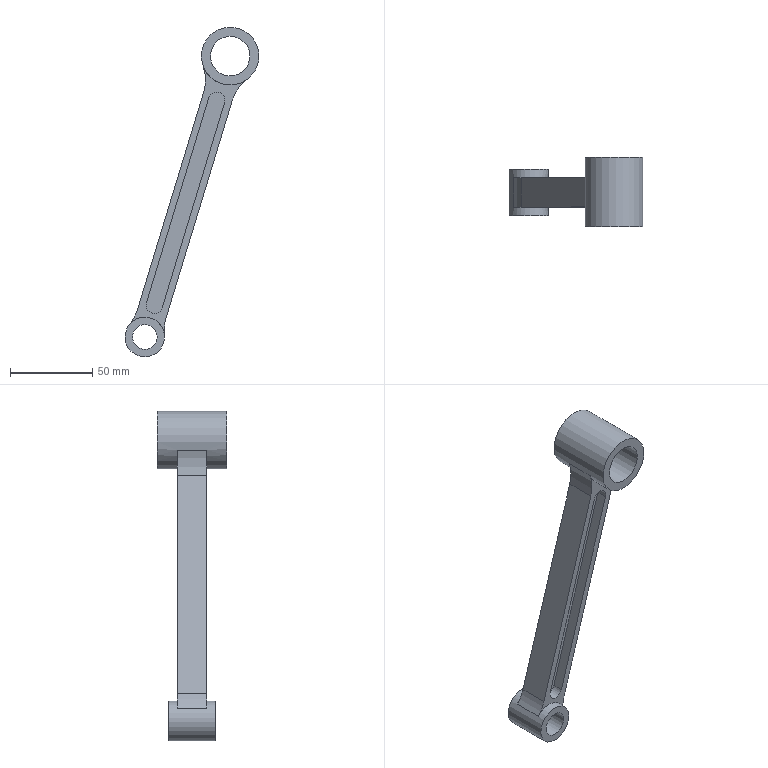Component | NX | ARTICULATE_ROD_3 | 1 solid | 26 faces | volume 60466 mm3 | plane 14 | cylinder 12 | commonest cylinder face diameters 48 x4 10 x4 24 x2 15 x1 35 x1